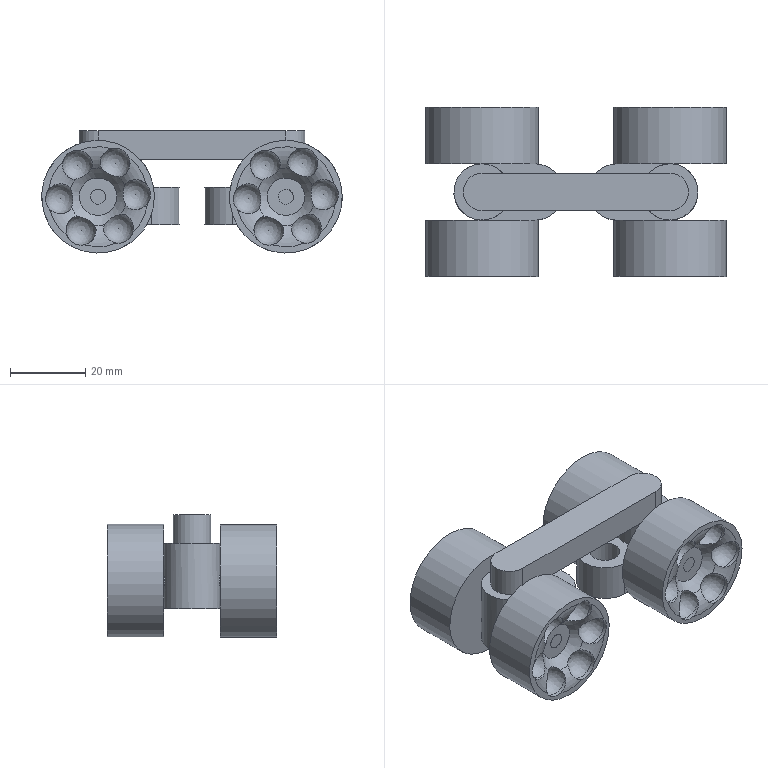Assembly | NX | mm | 7 component files | 7 solids | 132 faces | box 80 x 45 x 32.5 mm | volume 47813 mm3 | cylinder 48 | plane 32 | sphere 24 | torus 24 | cone 4 | commonest cylinder face diameters 8 x30 4 x8 15 x4 30 x4 10 x2
Bill of materials:
unnamed part 1 | 1 |  | Long, flat bar with an obround outline (straight sides, fully rounded ends). Two short cylindrical posts stick out from one face, one under each rounded end. The overall shape is a U or bridge, like a pull handle.
unnamed part 2 | 4 |  | Solid cylinder, like a thick disc, with a small hole bored through the center along its axis. The diameter is about twice the axial length.
unnamed part 3 | 2 |  | Obround plate (straight sides, rounded ends) with two through holes of about the same size, one near each rounded end. A taller cylindrical boss is built up around one of the holes, extending the bore. A thin cylindrical rod runs across the part, perpendicular to the plate's long axis and parallel to its faces. It passes through the boss and plate region and sticks out on both sides.
Mates:
1. concentric | rear_wheel 3 edge | steering_rod 2 arc
2. concentric | rear_wheel 2 edge | steering_rod 2 edge
3. concentric | steering_rod 1 edge | rear_wheel 1 edge
4. concentric | steering_rod 1 edge | rear_wheel 4 edge
5. concentric | steering_link 1 arc | steering_rod 2 edge
6. concentric | steering_link 1 arc | steering_rod 1 edge
7. distance | rear_wheel 2 face | rear_wheel 1 face